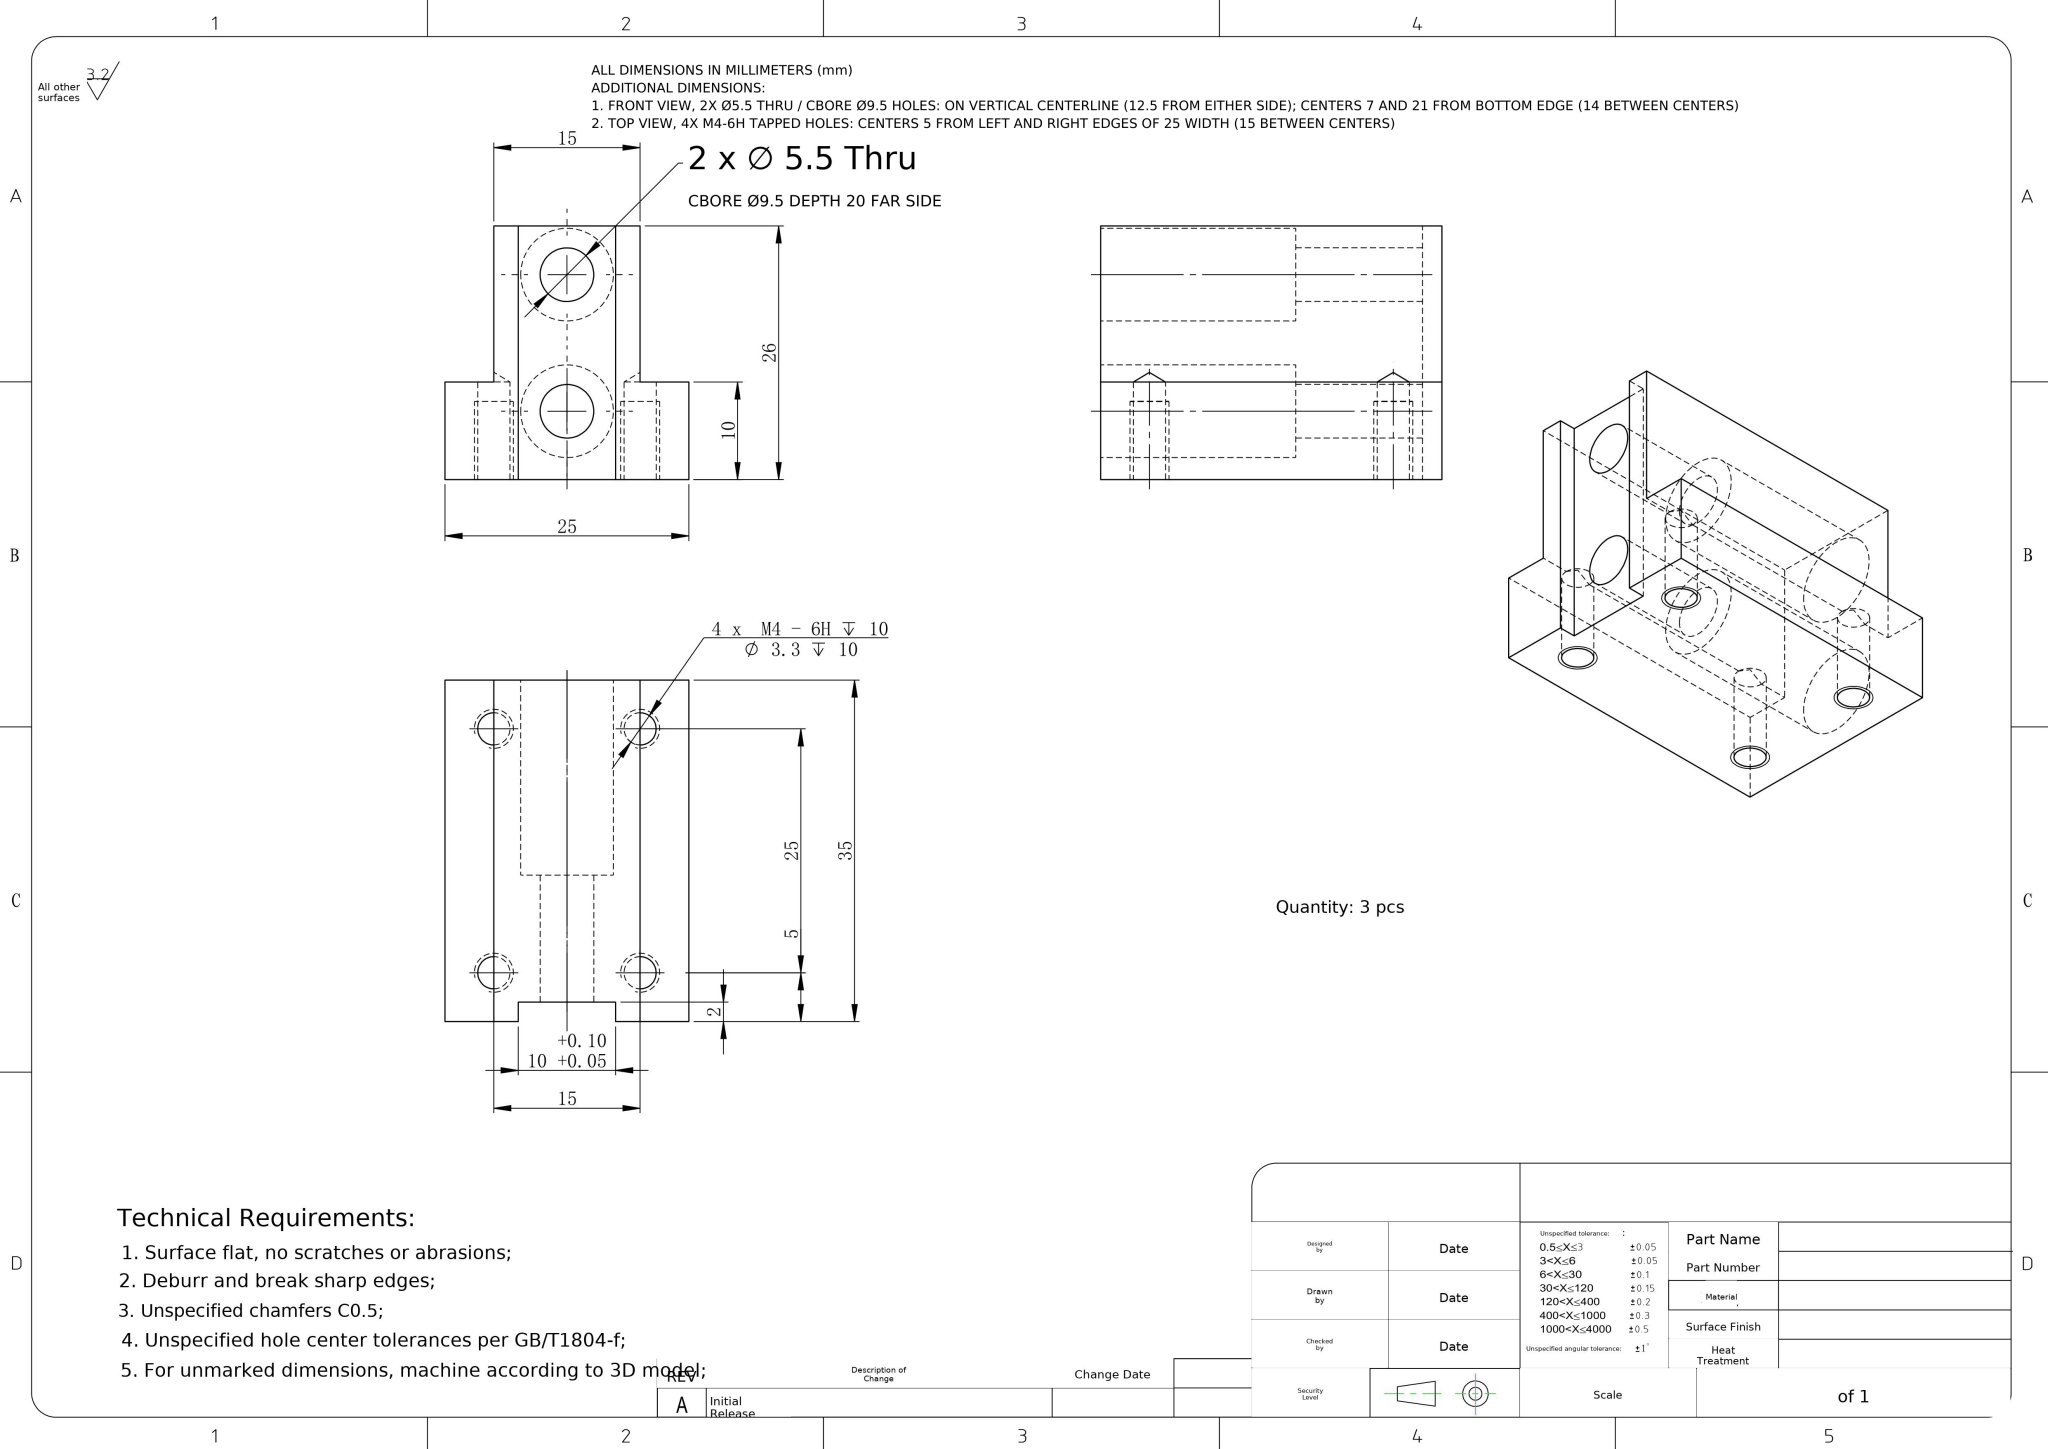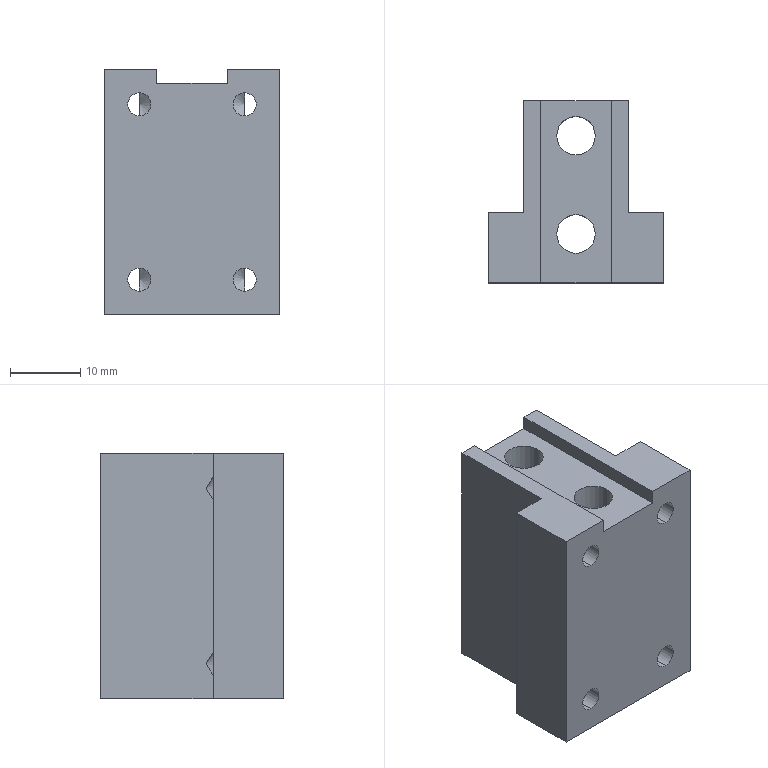Part | NX | mm | 1 solid | 36 faces | box 25 x 26 x 35 mm | volume 12829 mm3 | cylinder 16 | plane 16 | cone 4 | commonest cylinder face diameters 3.3 x8 9.5 x4 5.5 x4